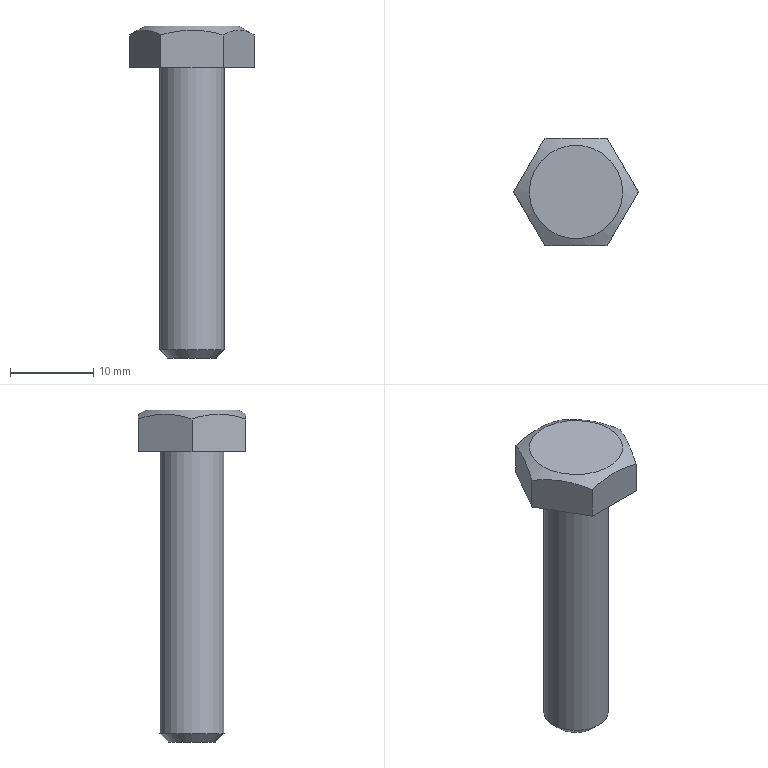Component | NX | BOLT_M8X35_2 | 1 solid | 12 faces | box 15.01 x 13 x 40 mm | volume 2369 mm3 | plane 9 | cone 2 | cylinder 1 | commonest cylinder face diameters 7.785 x1
STEP:
#1=CARTESIAN_POINT('',(0.,0.,0.));
#2=DIRECTION('',(0.,0.,1.));
#3=DIRECTION('',(1.,0.,0.));
#4=AXIS2_PLACEMENT_3D('',#1,#2,#3);
#5=CARTESIAN_POINT('',(4.607,42.,-63.5));
#6=VERTEX_POINT('',#5);
#7=CARTESIAN_POINT('',(7.5,42.,-63.5));
#8=DIRECTION('',(0.,0.,-1.));
#9=DIRECTION('',(-1.,0.,0.));
#10=AXIS2_PLACEMENT_3D('',#7,#8,#9);
#11=CIRCLE('',#10,2.893);
#12=CARTESIAN_POINT('',(7.5,42.,-63.5));
#13=DIRECTION('',(0.,0.,-1.));
#14=DIRECTION('',(-1.,0.,0.));
#15=AXIS2_PLACEMENT_3D('',#12,#13,#14);
#16=PLANE('',#15);
#17=CARTESIAN_POINT('',(0.,0.));
#18=DIRECTION('',(1.,0.));
#19=AXIS2_PLACEMENT_2D('',#17,#18);
#20=CIRCLE('',#19,2.893);
#21=(GEOMETRIC_REPRESENTATION_CONTEXT(2)PARAMETRIC_REPRESENTATION_CONTEXT()REPRESENTATION_CONTEXT('',''));
#22=DEFINITIONAL_REPRESENTATION('',(#20),#21);
#23=PCURVE('',#16,#22);
#24=CARTESIAN_POINT('',(7.5,42.,-62.5));
#25=DIRECTION('',(0.,0.,1.));
#26=DIRECTION('',(1.,0.,0.));
#27=AXIS2_PLACEMENT_3D('',#24,#25,#26);
#28=CONICAL_SURFACE('',#27,3.893,0.7854);
#29=CARTESIAN_POINT('',(9.425,-1.));
#30=DIRECTION('',(-1.,0.));
#31=VECTOR('',#30,1.);
#32=LINE('',#29,#31);
#33=(GEOMETRIC_REPRESENTATION_CONTEXT(2)PARAMETRIC_REPRESENTATION_CONTEXT()REPRESENTATION_CONTEXT('',''));
#34=DEFINITIONAL_REPRESENTATION('',(#32),#33);
#35=PCURVE('',#28,#34);
#36=SURFACE_CURVE('',#11,(#23,#35),.PCURVE_S1.);
#37=EDGE_CURVE('',#6,#6,#36,.T.);
#38=ORIENTED_EDGE('',*,*,#37,.T.);
#39=EDGE_LOOP('',(#38));
#40=FACE_BOUND('',#39,.T.);
#41=ADVANCED_FACE('',(#40),#16,.T.);
#42=CARTESIAN_POINT('',(3.607,42.,-62.5));
#43=VERTEX_POINT('',#42);
#44=CARTESIAN_POINT('',(11.393,42.,-62.5));
#45=VERTEX_POINT('',#44);
#46=CARTESIAN_POINT('',(7.5,42.,-62.5));
#47=DIRECTION('',(0.,0.,1.));
#48=DIRECTION('',(-1.,0.,0.));
#49=AXIS2_PLACEMENT_3D('',#46,#47,#48);
#50=CIRCLE('',#49,3.893);
#51=CARTESIAN_POINT('',(7.5,42.,-63.5));
#52=DIRECTION('',(0.,0.,1.));
#53=DIRECTION('',(1.,0.,0.));
#54=AXIS2_PLACEMENT_3D('',#51,#52,#53);
#55=CYLINDRICAL_SURFACE('',#54,3.893);
#56=CARTESIAN_POINT('',(3.142,1.));
#57=DIRECTION('',(1.,0.));
#58=VECTOR('',#57,1.);
#59=LINE('',#56,#58);
#60=(GEOMETRIC_REPRESENTATION_CONTEXT(2)PARAMETRIC_REPRESENTATION_CONTEXT()REPRESENTATION_CONTEXT('',''));
#61=DEFINITIONAL_REPRESENTATION('',(#59),#60);
#62=PCURVE('',#55,#61);
#63=CARTESIAN_POINT('',(3.142,0.));
#64=DIRECTION('',(1.,0.));
#65=VECTOR('',#64,1.);
#66=LINE('',#63,#65);
#67=(GEOMETRIC_REPRESENTATION_CONTEXT(2)PARAMETRIC_REPRESENTATION_CONTEXT()REPRESENTATION_CONTEXT('',''));
#68=DEFINITIONAL_REPRESENTATION('',(#66),#67);
#69=PCURVE('',#28,#68);
#70=SURFACE_CURVE('',#50,(#62,#69),.PCURVE_S1.);
#71=EDGE_CURVE('',#43,#45,#70,.T.);
#72=ORIENTED_EDGE('',*,*,#71,.T.);
#73=CARTESIAN_POINT('',(11.393,42.,-28.5));
#74=VERTEX_POINT('',#73);
#75=CARTESIAN_POINT('',(11.393,42.,-62.5));
#76=CARTESIAN_POINT('',(11.393,42.,-28.5));
#77=B_SPLINE_CURVE_WITH_KNOTS('',1,(#75,#76),.UNSPECIFIED.,.F.,.F.,(2,2),(1.,35.),.PIECEWISE_BEZIER_KNOTS.);
#78=CARTESIAN_POINT('',(6.283,0.));
#79=DIRECTION('',(0.,1.));
#80=VECTOR('',#79,1.);
#81=LINE('',#78,#80);
#82=(GEOMETRIC_REPRESENTATION_CONTEXT(2)PARAMETRIC_REPRESENTATION_CONTEXT()REPRESENTATION_CONTEXT('',''));
#83=DEFINITIONAL_REPRESENTATION('',(#81),#82);
#84=PCURVE('',#55,#83);
#85=CARTESIAN_POINT('',(0.,0.));
#86=DIRECTION('',(0.,1.));
#87=VECTOR('',#86,1.);
#88=LINE('',#85,#87);
#89=(GEOMETRIC_REPRESENTATION_CONTEXT(2)PARAMETRIC_REPRESENTATION_CONTEXT()REPRESENTATION_CONTEXT('',''));
#90=DEFINITIONAL_REPRESENTATION('',(#88),#89);
#91=PCURVE('',#55,#90);
#92=SEAM_CURVE('',#77,(#84,#91),.PCURVE_S1.);
#93=EDGE_CURVE('',#45,#74,#92,.T.);
#94=ORIENTED_EDGE('',*,*,#93,.T.);
#95=CARTESIAN_POINT('',(7.5,42.,-28.5));
#96=DIRECTION('',(0.,0.,-1.));
#97=DIRECTION('',(1.,0.,0.));
#98=AXIS2_PLACEMENT_3D('',#95,#96,#97);
#99=CIRCLE('',#98,3.893);
#100=CARTESIAN_POINT('',(6.283,35.));
#101=DIRECTION('',(-1.,0.));
#102=VECTOR('',#101,1.);
#103=LINE('',#100,#102);
#104=(GEOMETRIC_REPRESENTATION_CONTEXT(2)PARAMETRIC_REPRESENTATION_CONTEXT()REPRESENTATION_CONTEXT('',''));
#105=DEFINITIONAL_REPRESENTATION('',(#103),#104);
#106=PCURVE('',#55,#105);
#107=CARTESIAN_POINT('',(7.5,42.,-28.5));
#108=DIRECTION('',(0.,0.,-1.));
#109=DIRECTION('',(-1.,0.,0.));
#110=AXIS2_PLACEMENT_3D('',#107,#108,#109);
#111=PLANE('',#110);
#112=CARTESIAN_POINT('',(0.,0.));
#113=DIRECTION('',(-1.,0.));
#114=AXIS2_PLACEMENT_2D('',#112,#113);
#115=CIRCLE('',#114,3.893);
#116=(GEOMETRIC_REPRESENTATION_CONTEXT(2)PARAMETRIC_REPRESENTATION_CONTEXT()REPRESENTATION_CONTEXT('',''));
#117=DEFINITIONAL_REPRESENTATION('',(#115),#116);
#118=PCURVE('',#111,#117);
#119=SURFACE_CURVE('',#99,(#106,#118),.PCURVE_S1.);
#120=EDGE_CURVE('',#74,#74,#119,.T.);
#121=ORIENTED_EDGE('',*,*,#120,.T.);
#122=ORIENTED_EDGE('',*,*,#93,.F.);
#123=CARTESIAN_POINT('',(7.5,42.,-62.5));
#124=DIRECTION('',(0.,0.,1.));
#125=DIRECTION('',(-1.,0.,0.));
#126=AXIS2_PLACEMENT_3D('',#123,#124,#125);
#127=CIRCLE('',#126,3.893);
#128=CARTESIAN_POINT('',(-3.142,1.));
#129=DIRECTION('',(1.,0.));
#130=VECTOR('',#129,1.);
#131=LINE('',#128,#130);
#132=(GEOMETRIC_REPRESENTATION_CONTEXT(2)PARAMETRIC_REPRESENTATION_CONTEXT()REPRESENTATION_CONTEXT('',''));
#133=DEFINITIONAL_REPRESENTATION('',(#131),#132);
#134=PCURVE('',#55,#133);
#135=CARTESIAN_POINT('',(3.142,0.));
#136=DIRECTION('',(1.,-0.));
#137=VECTOR('',#136,1.);
#138=LINE('',#135,#137);
#139=(GEOMETRIC_REPRESENTATION_CONTEXT(2)PARAMETRIC_REPRESENTATION_CONTEXT()REPRESENTATION_CONTEXT('',''));
#140=DEFINITIONAL_REPRESENTATION('',(#138),#139);
#141=PCURVE('',#28,#140);
#142=SURFACE_CURVE('',#127,(#134,#141),.PCURVE_S1.);
#143=EDGE_CURVE('',#45,#43,#142,.T.);
#144=ORIENTED_EDGE('',*,*,#143,.T.);
#145=EDGE_LOOP('',(#72,#94,#121,#122,#144));
#146=FACE_BOUND('',#145,.T.);
#147=ADVANCED_FACE('',(#146),#55,.T.);
#148=CARTESIAN_POINT('',(15.006,42.,-24.583));
#149=VERTEX_POINT('',#148);
#150=CARTESIAN_POINT('',(11.253,48.5,-24.583));
#151=VERTEX_POINT('',#150);
#152=CARTESIAN_POINT('',(15.006,42.,-24.583));
#153=CARTESIAN_POINT('',(14.393,43.061,-24.23));
#154=CARTESIAN_POINT('',(13.771,44.139,-24.004));
#155=CARTESIAN_POINT('',(12.495,46.349,-24.002));
#156=CARTESIAN_POINT('',(11.866,47.437,-24.229));
#157=CARTESIAN_POINT('',(11.253,48.5,-24.583));
#158=B_SPLINE_CURVE_WITH_KNOTS('',3,(#152,#153,#154,#155,#156,#157),.UNSPECIFIED.,.F.,.F.,(4,2,4),(0.,0.5,1.),.UNSPECIFIED.);
#159=CARTESIAN_POINT('',(11.253,48.5,-23.5));
#160=DIRECTION('',(0.866,0.5,0.));
#161=DIRECTION('',(-0.5,0.866,0.));
#162=AXIS2_PLACEMENT_3D('',#159,#160,#161);
#163=PLANE('',#162);
#164=CARTESIAN_POINT('',(-7.506,-1.083));
#165=CARTESIAN_POINT('',(-6.28,-0.7296));
#166=CARTESIAN_POINT('',(-5.036,-0.5036));
#167=CARTESIAN_POINT('',(-2.484,-0.502));
#168=CARTESIAN_POINT('',(-1.227,-0.7291));
#169=CARTESIAN_POINT('',(0.,-1.083));
#170=B_SPLINE_CURVE_WITH_KNOTS('',3,(#164,#165,#166,#167,#168,#169),.UNSPECIFIED.,.F.,.F.,(4,2,4),(0.,0.5,1.),.UNSPECIFIED.);
#171=(GEOMETRIC_REPRESENTATION_CONTEXT(2)PARAMETRIC_REPRESENTATION_CONTEXT()REPRESENTATION_CONTEXT('',''));
#172=DEFINITIONAL_REPRESENTATION('',(#170),#171);
#173=PCURVE('',#163,#172);
#174=CARTESIAN_POINT('',(7.5,42.,-23.5));
#175=DIRECTION('',(0.,0.,-1.));
#176=DIRECTION('',(-1.,0.,0.));
#177=AXIS2_PLACEMENT_3D('',#174,#175,#176);
#178=CONICAL_SURFACE('',#177,5.629,1.047);
#179=CARTESIAN_POINT('',(3.142,1.083));
#180=CARTESIAN_POINT('',(3.129,1.051));
#181=CARTESIAN_POINT('',(3.102,0.9889));
#182=CARTESIAN_POINT('',(3.061,0.9022));
#183=CARTESIAN_POINT('',(3.018,0.8227));
#184=CARTESIAN_POINT('',(2.973,0.7508));
#185=CARTESIAN_POINT('',(2.926,0.6871));
#186=CARTESIAN_POINT('',(2.878,0.632));
#187=CARTESIAN_POINT('',(2.828,0.586));
#188=CARTESIAN_POINT('',(2.777,0.5495));
#189=CARTESIAN_POINT('',(2.725,0.5229));
#190=CARTESIAN_POINT('',(2.673,0.5066));
#191=CARTESIAN_POINT('',(2.619,0.501));
#192=CARTESIAN_POINT('',(2.566,0.5062));
#193=CARTESIAN_POINT('',(2.513,0.5221));
#194=CARTESIAN_POINT('',(2.46,0.5484));
#195=CARTESIAN_POINT('',(2.409,0.5848));
#196=CARTESIAN_POINT('',(2.359,0.6308));
#197=CARTESIAN_POINT('',(2.311,0.686));
#198=CARTESIAN_POINT('',(2.264,0.7499));
#199=CARTESIAN_POINT('',(2.218,0.822));
#200=CARTESIAN_POINT('',(2.175,0.9018));
#201=CARTESIAN_POINT('',(2.134,0.9888));
#202=CARTESIAN_POINT('',(2.107,1.051));
#203=CARTESIAN_POINT('',(2.094,1.083));
#204=B_SPLINE_CURVE_WITH_KNOTS('',3,(#179,#180,#181,#182,#183,#184,#185,#186,#187,#188,#189,#190,#191,#192,#193,#194,#195,#196,#197,#198,#199,#200,#201,#202,#203),.UNSPECIFIED.,.F.,.F.,(4,1,1,1,1,1,1,1,1,1,1,1,1,1,1,1,1,1,1,1,1,1,4),(0.,0.04545,0.09091,0.1364,0.1818,0.2273,0.2727,0.3182,0.3636,0.4091,0.4545,0.5,0.5455,0.5909,0.6364,0.6818,0.7273,0.7727,0.8182,0.8636,0.9091,0.9545,1.),.QUASI_UNIFORM_KNOTS.);
#205=(GEOMETRIC_REPRESENTATION_CONTEXT(2)PARAMETRIC_REPRESENTATION_CONTEXT()REPRESENTATION_CONTEXT('',''));
#206=DEFINITIONAL_REPRESENTATION('',(#204),#205);
#207=PCURVE('',#178,#206);
#208=SURFACE_CURVE('',#158,(#173,#207),.PCURVE_S1.);
#209=EDGE_CURVE('',#149,#151,#208,.T.);
#210=ORIENTED_EDGE('',*,*,#209,.F.);
#211=CARTESIAN_POINT('',(15.006,42.,-28.5));
#212=VERTEX_POINT('',#211);
#213=CARTESIAN_POINT('',(15.006,42.,-23.5));
#214=DIRECTION('',(0.,0.,-1.));
#215=VECTOR('',#214,1.);
#216=LINE('',#213,#215);
#217=CARTESIAN_POINT('',(-7.506,0.));
#218=DIRECTION('',(0.,-1.));
#219=VECTOR('',#218,1.);
#220=LINE('',#217,#219);
#221=(GEOMETRIC_REPRESENTATION_CONTEXT(2)PARAMETRIC_REPRESENTATION_CONTEXT()REPRESENTATION_CONTEXT('',''));
#222=DEFINITIONAL_REPRESENTATION('',(#220),#221);
#223=PCURVE('',#163,#222);
#224=CARTESIAN_POINT('',(15.006,42.,-23.5));
#225=DIRECTION('',(0.866,-0.5,0.));
#226=DIRECTION('',(0.5,0.866,0.));
#227=AXIS2_PLACEMENT_3D('',#224,#225,#226);
#228=PLANE('',#227);
#229=CARTESIAN_POINT('',(0.,0.));
#230=DIRECTION('',(0.,-1.));
#231=VECTOR('',#230,1.);
#232=LINE('',#229,#231);
#233=(GEOMETRIC_REPRESENTATION_CONTEXT(2)PARAMETRIC_REPRESENTATION_CONTEXT()REPRESENTATION_CONTEXT('',''));
#234=DEFINITIONAL_REPRESENTATION('',(#232),#233);
#235=PCURVE('',#228,#234);
#236=SURFACE_CURVE('',#216,(#223,#235),.PCURVE_S1.);
#237=EDGE_CURVE('',#149,#212,#236,.T.);
#238=ORIENTED_EDGE('',*,*,#237,.T.);
#239=CARTESIAN_POINT('',(11.253,48.5,-28.5));
#240=VERTEX_POINT('',#239);
#241=CARTESIAN_POINT('',(11.253,48.5,-28.5));
#242=DIRECTION('',(0.5,-0.866,0.));
#243=VECTOR('',#242,1.);
#244=LINE('',#241,#243);
#245=CARTESIAN_POINT('',(0.,-5.));
#246=DIRECTION('',(-1.,0.));
#247=VECTOR('',#246,1.);
#248=LINE('',#245,#247);
#249=(GEOMETRIC_REPRESENTATION_CONTEXT(2)PARAMETRIC_REPRESENTATION_CONTEXT()REPRESENTATION_CONTEXT('',''));
#250=DEFINITIONAL_REPRESENTATION('',(#248),#249);
#251=PCURVE('',#163,#250);
#252=CARTESIAN_POINT('',(-3.753,6.5));
#253=DIRECTION('',(-0.5,-0.866));
#254=VECTOR('',#253,1.);
#255=LINE('',#252,#254);
#256=(GEOMETRIC_REPRESENTATION_CONTEXT(2)PARAMETRIC_REPRESENTATION_CONTEXT()REPRESENTATION_CONTEXT('',''));
#257=DEFINITIONAL_REPRESENTATION('',(#255),#256);
#258=PCURVE('',#111,#257);
#259=SURFACE_CURVE('',#244,(#251,#258),.PCURVE_S1.);
#260=EDGE_CURVE('',#240,#212,#259,.T.);
#261=ORIENTED_EDGE('',*,*,#260,.F.);
#262=CARTESIAN_POINT('',(11.253,48.5,-23.5));
#263=DIRECTION('',(0.,0.,-1.));
#264=VECTOR('',#263,1.);
#265=LINE('',#262,#264);
#266=CARTESIAN_POINT('',(0.,0.));
#267=DIRECTION('',(0.,-1.));
#268=VECTOR('',#267,1.);
#269=LINE('',#266,#268);
#270=(GEOMETRIC_REPRESENTATION_CONTEXT(2)PARAMETRIC_REPRESENTATION_CONTEXT()REPRESENTATION_CONTEXT('',''));
#271=DEFINITIONAL_REPRESENTATION('',(#269),#270);
#272=PCURVE('',#163,#271);
#273=CARTESIAN_POINT('',(3.747,48.5,-23.5));
#274=DIRECTION('',(0.,1.,0.));
#275=DIRECTION('',(0.,0.,1.));
#276=AXIS2_PLACEMENT_3D('',#273,#274,#275);
#277=PLANE('',#276);
#278=CARTESIAN_POINT('',(0.,7.506));
#279=DIRECTION('',(-1.,0.));
#280=VECTOR('',#279,1.);
#281=LINE('',#278,#280);
#282=(GEOMETRIC_REPRESENTATION_CONTEXT(2)PARAMETRIC_REPRESENTATION_CONTEXT()REPRESENTATION_CONTEXT('',''));
#283=DEFINITIONAL_REPRESENTATION('',(#281),#282);
#284=PCURVE('',#277,#283);
#285=SURFACE_CURVE('',#265,(#272,#284),.PCURVE_S1.);
#286=EDGE_CURVE('',#151,#240,#285,.T.);
#287=ORIENTED_EDGE('',*,*,#286,.F.);
#288=EDGE_LOOP('',(#210,#238,#261,#287));
#289=FACE_BOUND('',#288,.T.);
#290=ADVANCED_FACE('',(#289),#163,.T.);
#291=CARTESIAN_POINT('',(11.253,35.5,-24.583));
#292=VERTEX_POINT('',#291);
#293=CARTESIAN_POINT('',(11.253,35.5,-24.583));
#294=CARTESIAN_POINT('',(11.866,36.561,-24.23));
#295=CARTESIAN_POINT('',(12.487,37.639,-24.004));
#296=CARTESIAN_POINT('',(13.764,39.849,-24.002));
#297=CARTESIAN_POINT('',(14.392,40.937,-24.229));
#298=CARTESIAN_POINT('',(15.006,42.,-24.583));
#299=B_SPLINE_CURVE_WITH_KNOTS('',3,(#293,#294,#295,#296,#297,#298),.UNSPECIFIED.,.F.,.F.,(4,2,4),(0.,0.5,1.),.UNSPECIFIED.);
#300=CARTESIAN_POINT('',(-7.506,-1.083));
#301=CARTESIAN_POINT('',(-6.28,-0.7296));
#302=CARTESIAN_POINT('',(-5.036,-0.5036));
#303=CARTESIAN_POINT('',(-2.484,-0.502));
#304=CARTESIAN_POINT('',(-1.227,-0.7291));
#305=CARTESIAN_POINT('',(0.,-1.083));
#306=B_SPLINE_CURVE_WITH_KNOTS('',3,(#300,#301,#302,#303,#304,#305),.UNSPECIFIED.,.F.,.F.,(4,2,4),(0.,0.5,1.),.UNSPECIFIED.);
#307=(GEOMETRIC_REPRESENTATION_CONTEXT(2)PARAMETRIC_REPRESENTATION_CONTEXT()REPRESENTATION_CONTEXT('',''));
#308=DEFINITIONAL_REPRESENTATION('',(#306),#307);
#309=PCURVE('',#228,#308);
#310=CARTESIAN_POINT('',(4.189,1.083));
#311=CARTESIAN_POINT('',(4.176,1.051));
#312=CARTESIAN_POINT('',(4.15,0.9889));
#313=CARTESIAN_POINT('',(4.108,0.9022));
#314=CARTESIAN_POINT('',(4.065,0.8227));
#315=CARTESIAN_POINT('',(4.02,0.7508));
#316=CARTESIAN_POINT('',(3.974,0.6871));
#317=CARTESIAN_POINT('',(3.925,0.632));
#318=CARTESIAN_POINT('',(3.876,0.586));
#319=CARTESIAN_POINT('',(3.825,0.5495));
#320=CARTESIAN_POINT('',(3.773,0.5229));
#321=CARTESIAN_POINT('',(3.72,0.5066));
#322=CARTESIAN_POINT('',(3.666,0.501));
#323=CARTESIAN_POINT('',(3.613,0.5062));
#324=CARTESIAN_POINT('',(3.56,0.5221));
#325=CARTESIAN_POINT('',(3.507,0.5484));
#326=CARTESIAN_POINT('',(3.456,0.5848));
#327=CARTESIAN_POINT('',(3.406,0.6308));
#328=CARTESIAN_POINT('',(3.358,0.686));
#329=CARTESIAN_POINT('',(3.311,0.7499));
#330=CARTESIAN_POINT('',(3.266,0.822));
#331=CARTESIAN_POINT('',(3.222,0.9018));
#332=CARTESIAN_POINT('',(3.181,0.9888));
#333=CARTESIAN_POINT('',(3.154,1.051));
#334=CARTESIAN_POINT('',(3.142,1.083));
#335=B_SPLINE_CURVE_WITH_KNOTS('',3,(#310,#311,#312,#313,#314,#315,#316,#317,#318,#319,#320,#321,#322,#323,#324,#325,#326,#327,#328,#329,#330,#331,#332,#333,#334),.UNSPECIFIED.,.F.,.F.,(4,1,1,1,1,1,1,1,1,1,1,1,1,1,1,1,1,1,1,1,1,1,4),(0.,0.04545,0.09091,0.1364,0.1818,0.2273,0.2727,0.3182,0.3636,0.4091,0.4545,0.5,0.5455,0.5909,0.6364,0.6818,0.7273,0.7727,0.8182,0.8636,0.9091,0.9545,1.),.QUASI_UNIFORM_KNOTS.);
#336=(GEOMETRIC_REPRESENTATION_CONTEXT(2)PARAMETRIC_REPRESENTATION_CONTEXT()REPRESENTATION_CONTEXT('',''));
#337=DEFINITIONAL_REPRESENTATION('',(#335),#336);
#338=PCURVE('',#178,#337);
#339=SURFACE_CURVE('',#299,(#309,#338),.PCURVE_S1.);
#340=EDGE_CURVE('',#292,#149,#339,.T.);
#341=ORIENTED_EDGE('',*,*,#340,.F.);
#342=CARTESIAN_POINT('',(11.253,35.5,-28.5));
#343=VERTEX_POINT('',#342);
#344=CARTESIAN_POINT('',(11.253,35.5,-23.5));
#345=DIRECTION('',(0.,0.,-1.));
#346=VECTOR('',#345,1.);
#347=LINE('',#344,#346);
#348=CARTESIAN_POINT('',(-7.506,0.));
#349=DIRECTION('',(0.,-1.));
#350=VECTOR('',#349,1.);
#351=LINE('',#348,#350);
#352=(GEOMETRIC_REPRESENTATION_CONTEXT(2)PARAMETRIC_REPRESENTATION_CONTEXT()REPRESENTATION_CONTEXT('',''));
#353=DEFINITIONAL_REPRESENTATION('',(#351),#352);
#354=PCURVE('',#228,#353);
#355=CARTESIAN_POINT('',(11.253,35.5,-23.5));
#356=DIRECTION('',(-0.,-1.,0.));
#357=DIRECTION('',(1.,-0.,0.));
#358=AXIS2_PLACEMENT_3D('',#355,#356,#357);
#359=PLANE('',#358);
#360=CARTESIAN_POINT('',(0.,0.));
#361=DIRECTION('',(0.,-1.));
#362=VECTOR('',#361,1.);
#363=LINE('',#360,#362);
#364=(GEOMETRIC_REPRESENTATION_CONTEXT(2)PARAMETRIC_REPRESENTATION_CONTEXT()REPRESENTATION_CONTEXT('',''));
#365=DEFINITIONAL_REPRESENTATION('',(#363),#364);
#366=PCURVE('',#359,#365);
#367=SURFACE_CURVE('',#347,(#354,#366),.PCURVE_S1.);
#368=EDGE_CURVE('',#292,#343,#367,.T.);
#369=ORIENTED_EDGE('',*,*,#368,.T.);
#370=CARTESIAN_POINT('',(15.006,42.,-28.5));
#371=DIRECTION('',(-0.5,-0.866,0.));
#372=VECTOR('',#371,1.);
#373=LINE('',#370,#372);
#374=CARTESIAN_POINT('',(0.,-5.));
#375=DIRECTION('',(-1.,0.));
#376=VECTOR('',#375,1.);
#377=LINE('',#374,#376);
#378=(GEOMETRIC_REPRESENTATION_CONTEXT(2)PARAMETRIC_REPRESENTATION_CONTEXT()REPRESENTATION_CONTEXT('',''));
#379=DEFINITIONAL_REPRESENTATION('',(#377),#378);
#380=PCURVE('',#228,#379);
#381=CARTESIAN_POINT('',(-7.506,0.));
#382=DIRECTION('',(0.5,-0.866));
#383=VECTOR('',#382,1.);
#384=LINE('',#381,#383);
#385=(GEOMETRIC_REPRESENTATION_CONTEXT(2)PARAMETRIC_REPRESENTATION_CONTEXT()REPRESENTATION_CONTEXT('',''));
#386=DEFINITIONAL_REPRESENTATION('',(#384),#385);
#387=PCURVE('',#111,#386);
#388=SURFACE_CURVE('',#373,(#380,#387),.PCURVE_S1.);
#389=EDGE_CURVE('',#212,#343,#388,.T.);
#390=ORIENTED_EDGE('',*,*,#389,.F.);
#391=ORIENTED_EDGE('',*,*,#237,.F.);
#392=EDGE_LOOP('',(#341,#369,#390,#391));
#393=FACE_BOUND('',#392,.T.);
#394=ADVANCED_FACE('',(#393),#228,.T.);
#395=CARTESIAN_POINT('',(3.747,35.5,-24.583));
#396=VERTEX_POINT('',#395);
#397=CARTESIAN_POINT('',(3.747,35.5,-24.583));
#398=CARTESIAN_POINT('',(4.968,35.5,-24.231));
#399=CARTESIAN_POINT('',(6.233,35.5,-24.003));
#400=CARTESIAN_POINT('',(8.769,35.5,-24.003));
#401=CARTESIAN_POINT('',(10.04,35.5,-24.233));
#402=CARTESIAN_POINT('',(11.253,35.5,-24.583));
#403=B_SPLINE_CURVE_WITH_KNOTS('',3,(#397,#398,#399,#400,#401,#402),.UNSPECIFIED.,.F.,.F.,(4,2,4),(0.,0.5,1.),.UNSPECIFIED.);
#404=CARTESIAN_POINT('',(-7.506,-1.083));
#405=CARTESIAN_POINT('',(-6.285,-0.731));
#406=CARTESIAN_POINT('',(-5.02,-0.5027));
#407=CARTESIAN_POINT('',(-2.483,-0.5029));
#408=CARTESIAN_POINT('',(-1.213,-0.7331));
#409=CARTESIAN_POINT('',(0.,-1.083));
#410=B_SPLINE_CURVE_WITH_KNOTS('',3,(#404,#405,#406,#407,#408,#409),.UNSPECIFIED.,.F.,.F.,(4,2,4),(0.,0.5,1.),.UNSPECIFIED.);
#411=(GEOMETRIC_REPRESENTATION_CONTEXT(2)PARAMETRIC_REPRESENTATION_CONTEXT()REPRESENTATION_CONTEXT('',''));
#412=DEFINITIONAL_REPRESENTATION('',(#410),#411);
#413=PCURVE('',#359,#412);
#414=CARTESIAN_POINT('',(5.236,1.083));
#415=CARTESIAN_POINT('',(5.223,1.051));
#416=CARTESIAN_POINT('',(5.197,0.9892));
#417=CARTESIAN_POINT('',(5.156,0.9025));
#418=CARTESIAN_POINT('',(5.112,0.8227));
#419=CARTESIAN_POINT('',(5.067,0.7506));
#420=CARTESIAN_POINT('',(5.02,0.6866));
#421=CARTESIAN_POINT('',(4.972,0.6313));
#422=CARTESIAN_POINT('',(4.922,0.5852));
#423=CARTESIAN_POINT('',(4.87,0.5488));
#424=CARTESIAN_POINT('',(4.818,0.5224));
#425=CARTESIAN_POINT('',(4.765,0.5063));
#426=CARTESIAN_POINT('',(4.712,0.501));
#427=CARTESIAN_POINT('',(4.659,0.5064));
#428=CARTESIAN_POINT('',(4.606,0.5225));
#429=CARTESIAN_POINT('',(4.554,0.5491));
#430=CARTESIAN_POINT('',(4.503,0.5857));
#431=CARTESIAN_POINT('',(4.453,0.6319));
#432=CARTESIAN_POINT('',(4.404,0.6874));
#433=CARTESIAN_POINT('',(4.357,0.7514));
#434=CARTESIAN_POINT('',(4.312,0.8236));
#435=CARTESIAN_POINT('',(4.269,0.9032));
#436=CARTESIAN_POINT('',(4.228,0.9897));
#437=CARTESIAN_POINT('',(4.202,1.051));
#438=CARTESIAN_POINT('',(4.189,1.083));
#439=B_SPLINE_CURVE_WITH_KNOTS('',3,(#414,#415,#416,#417,#418,#419,#420,#421,#422,#423,#424,#425,#426,#427,#428,#429,#430,#431,#432,#433,#434,#435,#436,#437,#438),.UNSPECIFIED.,.F.,.F.,(4,1,1,1,1,1,1,1,1,1,1,1,1,1,1,1,1,1,1,1,1,1,4),(0.,0.04545,0.09091,0.1364,0.1818,0.2273,0.2727,0.3182,0.3636,0.4091,0.4545,0.5,0.5455,0.5909,0.6364,0.6818,0.7273,0.7727,0.8182,0.8636,0.9091,0.9545,1.),.QUASI_UNIFORM_KNOTS.);
#440=(GEOMETRIC_REPRESENTATION_CONTEXT(2)PARAMETRIC_REPRESENTATION_CONTEXT()REPRESENTATION_CONTEXT('',''));
#441=DEFINITIONAL_REPRESENTATION('',(#439),#440);
#442=PCURVE('',#178,#441);
#443=SURFACE_CURVE('',#403,(#413,#442),.PCURVE_S1.);
#444=EDGE_CURVE('',#396,#292,#443,.T.);
#445=ORIENTED_EDGE('',*,*,#444,.F.);
#446=CARTESIAN_POINT('',(3.747,35.5,-28.5));
#447=VERTEX_POINT('',#446);
#448=CARTESIAN_POINT('',(3.747,35.5,-23.5));
#449=DIRECTION('',(0.,0.,-1.));
#450=VECTOR('',#449,1.);
#451=LINE('',#448,#450);
#452=CARTESIAN_POINT('',(-7.506,0.));
#453=DIRECTION('',(0.,-1.));
#454=VECTOR('',#453,1.);
#455=LINE('',#452,#454);
#456=(GEOMETRIC_REPRESENTATION_CONTEXT(2)PARAMETRIC_REPRESENTATION_CONTEXT()REPRESENTATION_CONTEXT('',''));
#457=DEFINITIONAL_REPRESENTATION('',(#455),#456);
#458=PCURVE('',#359,#457);
#459=CARTESIAN_POINT('',(3.747,35.5,-23.5));
#460=DIRECTION('',(-0.866,-0.5,0.));
#461=DIRECTION('',(0.5,-0.866,0.));
#462=AXIS2_PLACEMENT_3D('',#459,#460,#461);
#463=PLANE('',#462);
#464=CARTESIAN_POINT('',(0.,0.));
#465=DIRECTION('',(0.,-1.));
#466=VECTOR('',#465,1.);
#467=LINE('',#464,#466);
#468=(GEOMETRIC_REPRESENTATION_CONTEXT(2)PARAMETRIC_REPRESENTATION_CONTEXT()REPRESENTATION_CONTEXT('',''));
#469=DEFINITIONAL_REPRESENTATION('',(#467),#468);
#470=PCURVE('',#463,#469);
#471=SURFACE_CURVE('',#451,(#458,#470),.PCURVE_S1.);
#472=EDGE_CURVE('',#396,#447,#471,.T.);
#473=ORIENTED_EDGE('',*,*,#472,.T.);
#474=CARTESIAN_POINT('',(11.253,35.5,-28.5));
#475=DIRECTION('',(-1.,0.,0.));
#476=VECTOR('',#475,1.);
#477=LINE('',#474,#476);
#478=CARTESIAN_POINT('',(0.,-5.));
#479=DIRECTION('',(-1.,0.));
#480=VECTOR('',#479,1.);
#481=LINE('',#478,#480);
#482=(GEOMETRIC_REPRESENTATION_CONTEXT(2)PARAMETRIC_REPRESENTATION_CONTEXT()REPRESENTATION_CONTEXT('',''));
#483=DEFINITIONAL_REPRESENTATION('',(#481),#482);
#484=PCURVE('',#359,#483);
#485=CARTESIAN_POINT('',(-3.753,-6.5));
#486=DIRECTION('',(1.,0.));
#487=VECTOR('',#486,1.);
#488=LINE('',#485,#487);
#489=(GEOMETRIC_REPRESENTATION_CONTEXT(2)PARAMETRIC_REPRESENTATION_CONTEXT()REPRESENTATION_CONTEXT('',''));
#490=DEFINITIONAL_REPRESENTATION('',(#488),#489);
#491=PCURVE('',#111,#490);
#492=SURFACE_CURVE('',#477,(#484,#491),.PCURVE_S1.);
#493=EDGE_CURVE('',#343,#447,#492,.T.);
#494=ORIENTED_EDGE('',*,*,#493,.F.);
#495=ORIENTED_EDGE('',*,*,#368,.F.);
#496=EDGE_LOOP('',(#445,#473,#494,#495));
#497=FACE_BOUND('',#496,.T.);
#498=ADVANCED_FACE('',(#497),#359,.T.);
#499=CARTESIAN_POINT('',(-0.005553,42.,-24.583));
#500=VERTEX_POINT('',#499);
#501=CARTESIAN_POINT('',(-0.005553,42.,-24.583));
#502=CARTESIAN_POINT('',(0.6072,40.939,-24.23));
#503=CARTESIAN_POINT('',(1.229,39.861,-24.004));
#504=CARTESIAN_POINT('',(2.505,37.651,-24.002));
#505=CARTESIAN_POINT('',(3.134,36.563,-24.229));
#506=CARTESIAN_POINT('',(3.747,35.5,-24.583));
#507=B_SPLINE_CURVE_WITH_KNOTS('',3,(#501,#502,#503,#504,#505,#506),.UNSPECIFIED.,.F.,.F.,(4,2,4),(0.,0.5,1.),.UNSPECIFIED.);
#508=CARTESIAN_POINT('',(-7.506,-1.083));
#509=CARTESIAN_POINT('',(-6.28,-0.7296));
#510=CARTESIAN_POINT('',(-5.036,-0.5036));
#511=CARTESIAN_POINT('',(-2.484,-0.502));
#512=CARTESIAN_POINT('',(-1.227,-0.7291));
#513=CARTESIAN_POINT('',(0.,-1.083));
#514=B_SPLINE_CURVE_WITH_KNOTS('',3,(#508,#509,#510,#511,#512,#513),.UNSPECIFIED.,.F.,.F.,(4,2,4),(0.,0.5,1.),.UNSPECIFIED.);
#515=(GEOMETRIC_REPRESENTATION_CONTEXT(2)PARAMETRIC_REPRESENTATION_CONTEXT()REPRESENTATION_CONTEXT('',''));
#516=DEFINITIONAL_REPRESENTATION('',(#514),#515);
#517=PCURVE('',#463,#516);
#518=CARTESIAN_POINT('',(6.283,1.083));
#519=CARTESIAN_POINT('',(6.27,1.051));
#520=CARTESIAN_POINT('',(6.244,0.9889));
#521=CARTESIAN_POINT('',(6.203,0.9022));
#522=CARTESIAN_POINT('',(6.16,0.8227));
#523=CARTESIAN_POINT('',(6.115,0.7508));
#524=CARTESIAN_POINT('',(6.068,0.6871));
#525=CARTESIAN_POINT('',(6.02,0.632));
#526=CARTESIAN_POINT('',(5.97,0.586));
#527=CARTESIAN_POINT('',(5.919,0.5495));
#528=CARTESIAN_POINT('',(5.867,0.5229));
#529=CARTESIAN_POINT('',(5.814,0.5066));
#530=CARTESIAN_POINT('',(5.761,0.501));
#531=CARTESIAN_POINT('',(5.707,0.5062));
#532=CARTESIAN_POINT('',(5.654,0.5221));
#533=CARTESIAN_POINT('',(5.602,0.5484));
#534=CARTESIAN_POINT('',(5.551,0.5848));
#535=CARTESIAN_POINT('',(5.501,0.6308));
#536=CARTESIAN_POINT('',(5.452,0.686));
#537=CARTESIAN_POINT('',(5.405,0.7499));
#538=CARTESIAN_POINT('',(5.36,0.822));
#539=CARTESIAN_POINT('',(5.317,0.9018));
#540=CARTESIAN_POINT('',(5.275,0.9888));
#541=CARTESIAN_POINT('',(5.249,1.051));
#542=CARTESIAN_POINT('',(5.236,1.083));
#543=B_SPLINE_CURVE_WITH_KNOTS('',3,(#518,#519,#520,#521,#522,#523,#524,#525,#526,#527,#528,#529,#530,#531,#532,#533,#534,#535,#536,#537,#538,#539,#540,#541,#542),.UNSPECIFIED.,.F.,.F.,(4,1,1,1,1,1,1,1,1,1,1,1,1,1,1,1,1,1,1,1,1,1,4),(0.,0.04545,0.09091,0.1364,0.1818,0.2273,0.2727,0.3182,0.3636,0.4091,0.4545,0.5,0.5455,0.5909,0.6364,0.6818,0.7273,0.7727,0.8182,0.8636,0.9091,0.9545,1.),.QUASI_UNIFORM_KNOTS.);
#544=(GEOMETRIC_REPRESENTATION_CONTEXT(2)PARAMETRIC_REPRESENTATION_CONTEXT()REPRESENTATION_CONTEXT('',''));
#545=DEFINITIONAL_REPRESENTATION('',(#543),#544);
#546=PCURVE('',#178,#545);
#547=SURFACE_CURVE('',#507,(#517,#546),.PCURVE_S1.);
#548=EDGE_CURVE('',#500,#396,#547,.T.);
#549=ORIENTED_EDGE('',*,*,#548,.F.);
#550=CARTESIAN_POINT('',(-0.005553,42.,-28.5));
#551=VERTEX_POINT('',#550);
#552=CARTESIAN_POINT('',(-0.005553,42.,-23.5));
#553=DIRECTION('',(0.,0.,-1.));
#554=VECTOR('',#553,1.);
#555=LINE('',#552,#554);
#556=CARTESIAN_POINT('',(-7.506,0.));
#557=DIRECTION('',(0.,-1.));
#558=VECTOR('',#557,1.);
#559=LINE('',#556,#558);
#560=(GEOMETRIC_REPRESENTATION_CONTEXT(2)PARAMETRIC_REPRESENTATION_CONTEXT()REPRESENTATION_CONTEXT('',''));
#561=DEFINITIONAL_REPRESENTATION('',(#559),#560);
#562=PCURVE('',#463,#561);
#563=CARTESIAN_POINT('',(-0.005553,42.,-23.5));
#564=DIRECTION('',(-0.866,0.5,0.));
#565=DIRECTION('',(-0.5,-0.866,0.));
#566=AXIS2_PLACEMENT_3D('',#563,#564,#565);
#567=PLANE('',#566);
#568=CARTESIAN_POINT('',(-0.,0.));
#569=DIRECTION('',(0.,-1.));
#570=VECTOR('',#569,1.);
#571=LINE('',#568,#570);
#572=(GEOMETRIC_REPRESENTATION_CONTEXT(2)PARAMETRIC_REPRESENTATION_CONTEXT()REPRESENTATION_CONTEXT('',''));
#573=DEFINITIONAL_REPRESENTATION('',(#571),#572);
#574=PCURVE('',#567,#573);
#575=SURFACE_CURVE('',#555,(#562,#574),.PCURVE_S1.);
#576=EDGE_CURVE('',#500,#551,#575,.T.);
#577=ORIENTED_EDGE('',*,*,#576,.T.);
#578=CARTESIAN_POINT('',(3.747,35.5,-28.5));
#579=DIRECTION('',(-0.5,0.866,0.));
#580=VECTOR('',#579,1.);
#581=LINE('',#578,#580);
#582=CARTESIAN_POINT('',(0.,-5.));
#583=DIRECTION('',(-1.,0.));
#584=VECTOR('',#583,1.);
#585=LINE('',#582,#584);
#586=(GEOMETRIC_REPRESENTATION_CONTEXT(2)PARAMETRIC_REPRESENTATION_CONTEXT()REPRESENTATION_CONTEXT('',''));
#587=DEFINITIONAL_REPRESENTATION('',(#585),#586);
#588=PCURVE('',#463,#587);
#589=CARTESIAN_POINT('',(3.753,-6.5));
#590=DIRECTION('',(0.5,0.866));
#591=VECTOR('',#590,1.);
#592=LINE('',#589,#591);
#593=(GEOMETRIC_REPRESENTATION_CONTEXT(2)PARAMETRIC_REPRESENTATION_CONTEXT()REPRESENTATION_CONTEXT('',''));
#594=DEFINITIONAL_REPRESENTATION('',(#592),#593);
#595=PCURVE('',#111,#594);
#596=SURFACE_CURVE('',#581,(#588,#595),.PCURVE_S1.);
#597=EDGE_CURVE('',#447,#551,#596,.T.);
#598=ORIENTED_EDGE('',*,*,#597,.F.);
#599=ORIENTED_EDGE('',*,*,#472,.F.);
#600=EDGE_LOOP('',(#549,#577,#598,#599));
#601=FACE_BOUND('',#600,.T.);
#602=ADVANCED_FACE('',(#601),#463,.T.);
#603=CARTESIAN_POINT('',(3.747,48.5,-24.583));
#604=VERTEX_POINT('',#603);
#605=CARTESIAN_POINT('',(3.747,48.5,-24.583));
#606=CARTESIAN_POINT('',(3.134,47.439,-24.23));
#607=CARTESIAN_POINT('',(2.513,46.361,-24.004));
#608=CARTESIAN_POINT('',(1.236,44.151,-24.002));
#609=CARTESIAN_POINT('',(0.608,43.063,-24.229));
#610=CARTESIAN_POINT('',(-0.005553,42.,-24.583));
#611=B_SPLINE_CURVE_WITH_KNOTS('',3,(#605,#606,#607,#608,#609,#610),.UNSPECIFIED.,.F.,.F.,(4,2,4),(0.,0.5,1.),.UNSPECIFIED.);
#612=CARTESIAN_POINT('',(-7.506,-1.083));
#613=CARTESIAN_POINT('',(-6.28,-0.7296));
#614=CARTESIAN_POINT('',(-5.036,-0.5036));
#615=CARTESIAN_POINT('',(-2.484,-0.502));
#616=CARTESIAN_POINT('',(-1.227,-0.7291));
#617=CARTESIAN_POINT('',(0.,-1.083));
#618=B_SPLINE_CURVE_WITH_KNOTS('',3,(#612,#613,#614,#615,#616,#617),.UNSPECIFIED.,.F.,.F.,(4,2,4),(0.,0.5,1.),.UNSPECIFIED.);
#619=(GEOMETRIC_REPRESENTATION_CONTEXT(2)PARAMETRIC_REPRESENTATION_CONTEXT()REPRESENTATION_CONTEXT('',''));
#620=DEFINITIONAL_REPRESENTATION('',(#618),#619);
#621=PCURVE('',#567,#620);
#622=CARTESIAN_POINT('',(1.047,1.083));
#623=CARTESIAN_POINT('',(1.034,1.051));
#624=CARTESIAN_POINT('',(1.008,0.9889));
#625=CARTESIAN_POINT('',(0.9667,0.9022));
#626=CARTESIAN_POINT('',(0.9236,0.8227));
#627=CARTESIAN_POINT('',(0.8787,0.7508));
#628=CARTESIAN_POINT('',(0.832,0.6871));
#629=CARTESIAN_POINT('',(0.7838,0.632));
#630=CARTESIAN_POINT('',(0.7341,0.586));
#631=CARTESIAN_POINT('',(0.6831,0.5495));
#632=CARTESIAN_POINT('',(0.631,0.5229));
#633=CARTESIAN_POINT('',(0.5782,0.5066));
#634=CARTESIAN_POINT('',(0.5247,0.501));
#635=CARTESIAN_POINT('',(0.4712,0.5062));
#636=CARTESIAN_POINT('',(0.4182,0.5221));
#637=CARTESIAN_POINT('',(0.3659,0.5484));
#638=CARTESIAN_POINT('',(0.3147,0.5848));
#639=CARTESIAN_POINT('',(0.2647,0.6308));
#640=CARTESIAN_POINT('',(0.2161,0.686));
#641=CARTESIAN_POINT('',(0.1692,0.7499));
#642=CARTESIAN_POINT('',(0.124,0.822));
#643=CARTESIAN_POINT('',(0.0807,0.9018));
#644=CARTESIAN_POINT('',(0.03925,0.9888));
#645=CARTESIAN_POINT('',(0.01287,1.051));
#646=CARTESIAN_POINT('',(0.,1.083));
#647=B_SPLINE_CURVE_WITH_KNOTS('',3,(#622,#623,#624,#625,#626,#627,#628,#629,#630,#631,#632,#633,#634,#635,#636,#637,#638,#639,#640,#641,#642,#643,#644,#645,#646),.UNSPECIFIED.,.F.,.F.,(4,1,1,1,1,1,1,1,1,1,1,1,1,1,1,1,1,1,1,1,1,1,4),(0.,0.04545,0.09091,0.1364,0.1818,0.2273,0.2727,0.3182,0.3636,0.4091,0.4545,0.5,0.5455,0.5909,0.6364,0.6818,0.7273,0.7727,0.8182,0.8636,0.9091,0.9545,1.),.QUASI_UNIFORM_KNOTS.);
#648=(GEOMETRIC_REPRESENTATION_CONTEXT(2)PARAMETRIC_REPRESENTATION_CONTEXT()REPRESENTATION_CONTEXT('',''));
#649=DEFINITIONAL_REPRESENTATION('',(#647),#648);
#650=PCURVE('',#178,#649);
#651=SURFACE_CURVE('',#611,(#621,#650),.PCURVE_S1.);
#652=EDGE_CURVE('',#604,#500,#651,.T.);
#653=ORIENTED_EDGE('',*,*,#652,.F.);
#654=CARTESIAN_POINT('',(3.747,48.5,-28.5));
#655=VERTEX_POINT('',#654);
#656=CARTESIAN_POINT('',(3.747,48.5,-23.5));
#657=DIRECTION('',(0.,0.,-1.));
#658=VECTOR('',#657,1.);
#659=LINE('',#656,#658);
#660=CARTESIAN_POINT('',(-7.506,0.));
#661=DIRECTION('',(0.,-1.));
#662=VECTOR('',#661,1.);
#663=LINE('',#660,#662);
#664=(GEOMETRIC_REPRESENTATION_CONTEXT(2)PARAMETRIC_REPRESENTATION_CONTEXT()REPRESENTATION_CONTEXT('',''));
#665=DEFINITIONAL_REPRESENTATION('',(#663),#664);
#666=PCURVE('',#567,#665);
#667=CARTESIAN_POINT('',(0.,0.));
#668=DIRECTION('',(-1.,0.));
#669=VECTOR('',#668,1.);
#670=LINE('',#667,#669);
#671=(GEOMETRIC_REPRESENTATION_CONTEXT(2)PARAMETRIC_REPRESENTATION_CONTEXT()REPRESENTATION_CONTEXT('',''));
#672=DEFINITIONAL_REPRESENTATION('',(#670),#671);
#673=PCURVE('',#277,#672);
#674=SURFACE_CURVE('',#659,(#666,#673),.PCURVE_S1.);
#675=EDGE_CURVE('',#604,#655,#674,.T.);
#676=ORIENTED_EDGE('',*,*,#675,.T.);
#677=CARTESIAN_POINT('',(-0.005553,42.,-28.5));
#678=DIRECTION('',(0.5,0.866,0.));
#679=VECTOR('',#678,1.);
#680=LINE('',#677,#679);
#681=CARTESIAN_POINT('',(0.,-5.));
#682=DIRECTION('',(-1.,0.));
#683=VECTOR('',#682,1.);
#684=LINE('',#681,#683);
#685=(GEOMETRIC_REPRESENTATION_CONTEXT(2)PARAMETRIC_REPRESENTATION_CONTEXT()REPRESENTATION_CONTEXT('',''));
#686=DEFINITIONAL_REPRESENTATION('',(#684),#685);
#687=PCURVE('',#567,#686);
#688=CARTESIAN_POINT('',(7.506,0.));
#689=DIRECTION('',(-0.5,0.866));
#690=VECTOR('',#689,1.);
#691=LINE('',#688,#690);
#692=(GEOMETRIC_REPRESENTATION_CONTEXT(2)PARAMETRIC_REPRESENTATION_CONTEXT()REPRESENTATION_CONTEXT('',''));
#693=DEFINITIONAL_REPRESENTATION('',(#691),#692);
#694=PCURVE('',#111,#693);
#695=SURFACE_CURVE('',#680,(#687,#694),.PCURVE_S1.);
#696=EDGE_CURVE('',#551,#655,#695,.T.);
#697=ORIENTED_EDGE('',*,*,#696,.F.);
#698=ORIENTED_EDGE('',*,*,#576,.F.);
#699=EDGE_LOOP('',(#653,#676,#697,#698));
#700=FACE_BOUND('',#699,.T.);
#701=ADVANCED_FACE('',(#700),#567,.T.);
#702=CARTESIAN_POINT('',(11.253,48.5,-24.583));
#703=CARTESIAN_POINT('',(10.04,48.5,-24.233));
#704=CARTESIAN_POINT('',(8.769,48.5,-24.003));
#705=CARTESIAN_POINT('',(6.233,48.5,-24.003));
#706=CARTESIAN_POINT('',(4.968,48.5,-24.231));
#707=CARTESIAN_POINT('',(3.747,48.5,-24.583));
#708=B_SPLINE_CURVE_WITH_KNOTS('',3,(#702,#703,#704,#705,#706,#707),.UNSPECIFIED.,.F.,.F.,(4,2,4),(0.,0.5,1.),.UNSPECIFIED.);
#709=CARTESIAN_POINT('',(-1.083,7.506));
#710=CARTESIAN_POINT('',(-0.7331,6.292));
#711=CARTESIAN_POINT('',(-0.5029,5.022));
#712=CARTESIAN_POINT('',(-0.5027,2.486));
#713=CARTESIAN_POINT('',(-0.731,1.221));
#714=CARTESIAN_POINT('',(-1.083,-0.));
#715=B_SPLINE_CURVE_WITH_KNOTS('',3,(#709,#710,#711,#712,#713,#714),.UNSPECIFIED.,.F.,.F.,(4,2,4),(0.,0.5,1.),.UNSPECIFIED.);
#716=(GEOMETRIC_REPRESENTATION_CONTEXT(2)PARAMETRIC_REPRESENTATION_CONTEXT()REPRESENTATION_CONTEXT('',''));
#717=DEFINITIONAL_REPRESENTATION('',(#715),#716);
#718=PCURVE('',#277,#717);
#719=CARTESIAN_POINT('',(2.094,1.083));
#720=CARTESIAN_POINT('',(2.082,1.051));
#721=CARTESIAN_POINT('',(2.056,0.9897));
#722=CARTESIAN_POINT('',(2.014,0.9032));
#723=CARTESIAN_POINT('',(1.971,0.8236));
#724=CARTESIAN_POINT('',(1.926,0.7514));
#725=CARTESIAN_POINT('',(1.879,0.6874));
#726=CARTESIAN_POINT('',(1.831,0.6319));
#727=CARTESIAN_POINT('',(1.781,0.5857));
#728=CARTESIAN_POINT('',(1.729,0.5491));
#729=CARTESIAN_POINT('',(1.677,0.5225));
#730=CARTESIAN_POINT('',(1.624,0.5064));
#731=CARTESIAN_POINT('',(1.571,0.501));
#732=CARTESIAN_POINT('',(1.518,0.5063));
#733=CARTESIAN_POINT('',(1.465,0.5224));
#734=CARTESIAN_POINT('',(1.413,0.5488));
#735=CARTESIAN_POINT('',(1.362,0.5852));
#736=CARTESIAN_POINT('',(1.312,0.6313));
#737=CARTESIAN_POINT('',(1.263,0.6866));
#738=CARTESIAN_POINT('',(1.216,0.7506));
#739=CARTESIAN_POINT('',(1.171,0.8227));
#740=CARTESIAN_POINT('',(1.128,0.9025));
#741=CARTESIAN_POINT('',(1.086,0.9892));
#742=CARTESIAN_POINT('',(1.06,1.051));
#743=CARTESIAN_POINT('',(1.047,1.083));
#744=B_SPLINE_CURVE_WITH_KNOTS('',3,(#719,#720,#721,#722,#723,#724,#725,#726,#727,#728,#729,#730,#731,#732,#733,#734,#735,#736,#737,#738,#739,#740,#741,#742,#743),.UNSPECIFIED.,.F.,.F.,(4,1,1,1,1,1,1,1,1,1,1,1,1,1,1,1,1,1,1,1,1,1,4),(0.,0.04545,0.09091,0.1364,0.1818,0.2273,0.2727,0.3182,0.3636,0.4091,0.4545,0.5,0.5455,0.5909,0.6364,0.6818,0.7273,0.7727,0.8182,0.8636,0.9091,0.9545,1.),.QUASI_UNIFORM_KNOTS.);
#745=(GEOMETRIC_REPRESENTATION_CONTEXT(2)PARAMETRIC_REPRESENTATION_CONTEXT()REPRESENTATION_CONTEXT('',''));
#746=DEFINITIONAL_REPRESENTATION('',(#744),#745);
#747=PCURVE('',#178,#746);
#748=SURFACE_CURVE('',#708,(#718,#747),.PCURVE_S1.);
#749=EDGE_CURVE('',#151,#604,#748,.T.);
#750=ORIENTED_EDGE('',*,*,#749,.F.);
#751=ORIENTED_EDGE('',*,*,#286,.T.);
#752=CARTESIAN_POINT('',(3.747,48.5,-28.5));
#753=DIRECTION('',(1.,0.,0.));
#754=VECTOR('',#753,1.);
#755=LINE('',#752,#754);
#756=CARTESIAN_POINT('',(-5.,0.));
#757=DIRECTION('',(0.,1.));
#758=VECTOR('',#757,1.);
#759=LINE('',#756,#758);
#760=(GEOMETRIC_REPRESENTATION_CONTEXT(2)PARAMETRIC_REPRESENTATION_CONTEXT()REPRESENTATION_CONTEXT('',''));
#761=DEFINITIONAL_REPRESENTATION('',(#759),#760);
#762=PCURVE('',#277,#761);
#763=CARTESIAN_POINT('',(3.753,6.5));
#764=DIRECTION('',(-1.,0.));
#765=VECTOR('',#764,1.);
#766=LINE('',#763,#765);
#767=(GEOMETRIC_REPRESENTATION_CONTEXT(2)PARAMETRIC_REPRESENTATION_CONTEXT()REPRESENTATION_CONTEXT('',''));
#768=DEFINITIONAL_REPRESENTATION('',(#766),#767);
#769=PCURVE('',#111,#768);
#770=SURFACE_CURVE('',#755,(#762,#769),.PCURVE_S1.);
#771=EDGE_CURVE('',#655,#240,#770,.T.);
#772=ORIENTED_EDGE('',*,*,#771,.F.);
#773=ORIENTED_EDGE('',*,*,#675,.F.);
#774=EDGE_LOOP('',(#750,#751,#772,#773));
#775=FACE_BOUND('',#774,.T.);
#776=ADVANCED_FACE('',(#775),#277,.T.);
#777=ORIENTED_EDGE('',*,*,#120,.F.);
#778=EDGE_LOOP('',(#777));
#779=FACE_BOUND('',#778,.T.);
#780=ORIENTED_EDGE('',*,*,#260,.T.);
#781=ORIENTED_EDGE('',*,*,#389,.T.);
#782=ORIENTED_EDGE('',*,*,#493,.T.);
#783=ORIENTED_EDGE('',*,*,#597,.T.);
#784=ORIENTED_EDGE('',*,*,#696,.T.);
#785=ORIENTED_EDGE('',*,*,#771,.T.);
#786=EDGE_LOOP('',(#780,#781,#782,#783,#784,#785));
#787=FACE_BOUND('',#786,.T.);
#788=ADVANCED_FACE('',(#779,#787),#111,.T.);
#789=ORIENTED_EDGE('',*,*,#37,.F.);
#790=CARTESIAN_POINT('',(4.607,42.,-63.5));
#791=CARTESIAN_POINT('',(3.607,42.,-62.5));
#792=B_SPLINE_CURVE_WITH_KNOTS('',1,(#790,#791),.UNSPECIFIED.,.F.,.F.,(2,2),(-1.414,0.),.PIECEWISE_BEZIER_KNOTS.);
#793=CARTESIAN_POINT('',(9.425,0.));
#794=DIRECTION('',(0.,1.));
#795=VECTOR('',#794,1.);
#796=LINE('',#793,#795);
#797=(GEOMETRIC_REPRESENTATION_CONTEXT(2)PARAMETRIC_REPRESENTATION_CONTEXT()REPRESENTATION_CONTEXT('',''));
#798=DEFINITIONAL_REPRESENTATION('',(#796),#797);
#799=PCURVE('',#28,#798);
#800=CARTESIAN_POINT('',(3.142,0.));
#801=DIRECTION('',(0.,1.));
#802=VECTOR('',#801,1.);
#803=LINE('',#800,#802);
#804=(GEOMETRIC_REPRESENTATION_CONTEXT(2)PARAMETRIC_REPRESENTATION_CONTEXT()REPRESENTATION_CONTEXT('',''));
#805=DEFINITIONAL_REPRESENTATION('',(#803),#804);
#806=PCURVE('',#28,#805);
#807=SEAM_CURVE('',#792,(#799,#806),.PCURVE_S1.);
#808=EDGE_CURVE('',#6,#43,#807,.T.);
#809=ORIENTED_EDGE('',*,*,#808,.T.);
#810=ORIENTED_EDGE('',*,*,#143,.F.);
#811=ORIENTED_EDGE('',*,*,#71,.F.);
#812=ORIENTED_EDGE('',*,*,#808,.F.);
#813=EDGE_LOOP('',(#789,#809,#810,#811,#812));
#814=FACE_BOUND('',#813,.T.);
#815=ADVANCED_FACE('',(#814),#28,.T.);
#816=ORIENTED_EDGE('',*,*,#209,.T.);
#817=ORIENTED_EDGE('',*,*,#749,.T.);
#818=ORIENTED_EDGE('',*,*,#652,.T.);
#819=CARTESIAN_POINT('',(1.871,42.,-23.5));
#820=VERTEX_POINT('',#819);
#821=CARTESIAN_POINT('',(1.871,42.,-23.5));
#822=CARTESIAN_POINT('',(-0.005553,42.,-24.583));
#823=B_SPLINE_CURVE_WITH_KNOTS('',1,(#821,#822),.UNSPECIFIED.,.F.,.F.,(2,2),(0.,2.167),.PIECEWISE_BEZIER_KNOTS.);
#824=CARTESIAN_POINT('',(0.,0.));
#825=DIRECTION('',(0.,1.));
#826=VECTOR('',#825,1.);
#827=LINE('',#824,#826);
#828=(GEOMETRIC_REPRESENTATION_CONTEXT(2)PARAMETRIC_REPRESENTATION_CONTEXT()REPRESENTATION_CONTEXT('',''));
#829=DEFINITIONAL_REPRESENTATION('',(#827),#828);
#830=PCURVE('',#178,#829);
#831=CARTESIAN_POINT('',(6.283,0.));
#832=DIRECTION('',(0.,1.));
#833=VECTOR('',#832,1.);
#834=LINE('',#831,#833);
#835=(GEOMETRIC_REPRESENTATION_CONTEXT(2)PARAMETRIC_REPRESENTATION_CONTEXT()REPRESENTATION_CONTEXT('',''));
#836=DEFINITIONAL_REPRESENTATION('',(#834),#835);
#837=PCURVE('',#178,#836);
#838=SEAM_CURVE('',#823,(#830,#837),.PCURVE_S1.);
#839=EDGE_CURVE('',#820,#500,#838,.T.);
#840=ORIENTED_EDGE('',*,*,#839,.F.);
#841=CARTESIAN_POINT('',(7.5,42.,-23.5));
#842=DIRECTION('',(0.,0.,-1.));
#843=DIRECTION('',(-1.,0.,0.));
#844=AXIS2_PLACEMENT_3D('',#841,#842,#843);
#845=CIRCLE('',#844,5.629);
#846=CARTESIAN_POINT('',(0.,0.));
#847=DIRECTION('',(1.,0.));
#848=VECTOR('',#847,1.);
#849=LINE('',#846,#848);
#850=(GEOMETRIC_REPRESENTATION_CONTEXT(2)PARAMETRIC_REPRESENTATION_CONTEXT()REPRESENTATION_CONTEXT('',''));
#851=DEFINITIONAL_REPRESENTATION('',(#849),#850);
#852=PCURVE('',#178,#851);
#853=CARTESIAN_POINT('',(7.5,42.,-23.5));
#854=DIRECTION('',(0.,0.,-1.));
#855=DIRECTION('',(-1.,0.,0.));
#856=AXIS2_PLACEMENT_3D('',#853,#854,#855);
#857=PLANE('',#856);
#858=CARTESIAN_POINT('',(0.,0.));
#859=DIRECTION('',(1.,0.));
#860=AXIS2_PLACEMENT_2D('',#858,#859);
#861=CIRCLE('',#860,5.629);
#862=(GEOMETRIC_REPRESENTATION_CONTEXT(2)PARAMETRIC_REPRESENTATION_CONTEXT()REPRESENTATION_CONTEXT('',''));
#863=DEFINITIONAL_REPRESENTATION('',(#861),#862);
#864=PCURVE('',#857,#863);
#865=SURFACE_CURVE('',#845,(#852,#864),.PCURVE_S1.);
#866=EDGE_CURVE('',#820,#820,#865,.T.);
#867=ORIENTED_EDGE('',*,*,#866,.T.);
#868=ORIENTED_EDGE('',*,*,#839,.T.);
#869=ORIENTED_EDGE('',*,*,#548,.T.);
#870=ORIENTED_EDGE('',*,*,#444,.T.);
#871=ORIENTED_EDGE('',*,*,#340,.T.);
#872=EDGE_LOOP('',(#816,#817,#818,#840,#867,#868,#869,#870,#871));
#873=FACE_BOUND('',#872,.T.);
#874=ADVANCED_FACE('',(#873),#178,.T.);
#875=ORIENTED_EDGE('',*,*,#866,.F.);
#876=EDGE_LOOP('',(#875));
#877=FACE_BOUND('',#876,.T.);
#878=ADVANCED_FACE('',(#877),#857,.F.);
#879=CLOSED_SHELL('',(#41,#147,#290,#394,#498,#602,#701,#776,#788,#815,#874,#878));
#880=MANIFOLD_SOLID_BREP('',#879);
#881=(LENGTH_UNIT()NAMED_UNIT(*)SI_UNIT(.MILLI.,.METRE.));
#882=UNCERTAINTY_MEASURE_WITH_UNIT(LENGTH_MEASURE(0.0005),#881,'','');
#883=(NAMED_UNIT(*)PLANE_ANGLE_UNIT()SI_UNIT($,.RADIAN.));
#884=(NAMED_UNIT(*)SI_UNIT($,.STERADIAN.)SOLID_ANGLE_UNIT());
#885=(GEOMETRIC_REPRESENTATION_CONTEXT(3)GLOBAL_UNCERTAINTY_ASSIGNED_CONTEXT((#882))GLOBAL_UNIT_ASSIGNED_CONTEXT((#881,#883,#884))REPRESENTATION_CONTEXT('',''));
#886=ADVANCED_BREP_SHAPE_REPRESENTATION('',(#4,#880),#885);